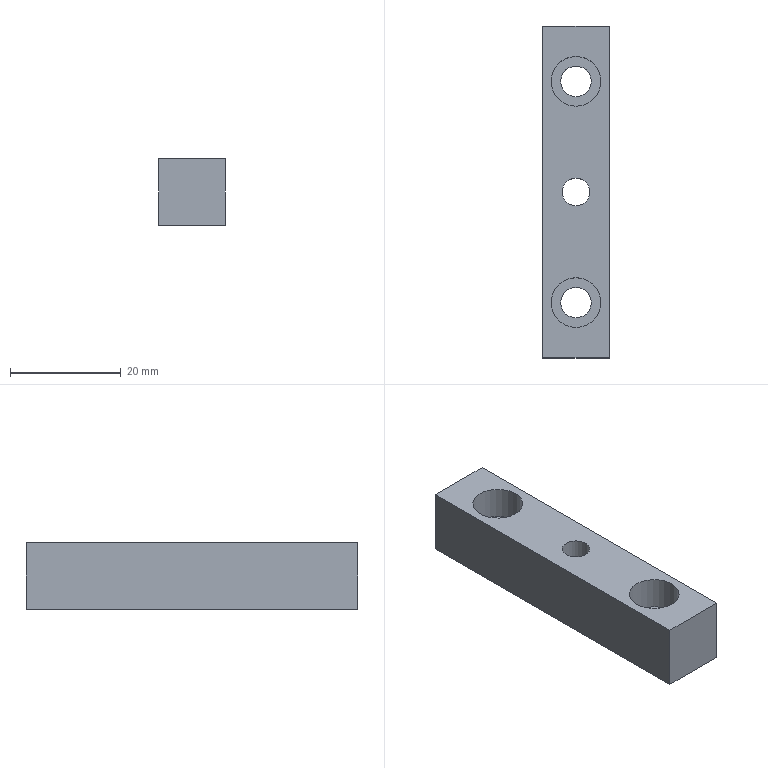Component | NX | COVER_PLATE | 1 solid | 13 faces | box 12 x 60 x 12 mm | volume 7356 mm3 | plane 8 | cylinder 5 | commonest cylinder face diameters 5.5 x2 9 x2 5 x1
STEP:
#1=CARTESIAN_POINT('',(0.,0.,0.));
#2=DIRECTION('',(0.,0.,1.));
#3=DIRECTION('',(1.,0.,0.));
#4=AXIS2_PLACEMENT_3D('',#1,#2,#3);
#5=CARTESIAN_POINT('',(0.,17.25,53.5));
#6=VERTEX_POINT('',#5);
#7=CARTESIAN_POINT('',(0.,20.,53.5));
#8=DIRECTION('',(0.,0.,-1.));
#9=DIRECTION('',(0.,-1.,0.));
#10=AXIS2_PLACEMENT_3D('',#7,#8,#9);
#11=CIRCLE('',#10,2.75);
#12=CARTESIAN_POINT('',(0.,20.,65.5));
#13=DIRECTION('',(0.,0.,-1.));
#14=DIRECTION('',(0.,1.,0.));
#15=AXIS2_PLACEMENT_3D('',#12,#13,#14);
#16=CYLINDRICAL_SURFACE('',#15,2.75);
#17=CARTESIAN_POINT('',(3.142,12.));
#18=DIRECTION('',(1.,0.));
#19=VECTOR('',#18,1.);
#20=LINE('',#17,#19);
#21=(GEOMETRIC_REPRESENTATION_CONTEXT(2)PARAMETRIC_REPRESENTATION_CONTEXT()REPRESENTATION_CONTEXT('',''));
#22=DEFINITIONAL_REPRESENTATION('',(#20),#21);
#23=PCURVE('',#16,#22);
#24=CARTESIAN_POINT('',(0.,-0.,53.5));
#25=DIRECTION('',(0.,0.,1.));
#26=DIRECTION('',(0.,-1.,0.));
#27=AXIS2_PLACEMENT_3D('',#24,#25,#26);
#28=PLANE('',#27);
#29=CARTESIAN_POINT('',(-17.25,-0.));
#30=CARTESIAN_POINT('',(-17.25,-4.763));
#31=CARTESIAN_POINT('',(-21.375,-2.382));
#32=CARTESIAN_POINT('',(-25.5,-0.));
#33=CARTESIAN_POINT('',(-21.375,2.382));
#34=CARTESIAN_POINT('',(-17.25,4.763));
#35=CARTESIAN_POINT('',(-17.25,-0.));
#36=(BOUNDED_CURVE()B_SPLINE_CURVE(2,(#29,#30,#31,#32,#33,#34,#35),.UNSPECIFIED.,.T.,.F.)B_SPLINE_CURVE_WITH_KNOTS((1,2,2,2,2,1),(-2.094,0.,2.094,4.189,6.283,8.378),.UNSPECIFIED.)CURVE()GEOMETRIC_REPRESENTATION_ITEM()RATIONAL_B_SPLINE_CURVE((1.,0.5,1.,0.5,1.,0.5,1.))REPRESENTATION_ITEM(''));
#37=(GEOMETRIC_REPRESENTATION_CONTEXT(2)PARAMETRIC_REPRESENTATION_CONTEXT()REPRESENTATION_CONTEXT('',''));
#38=DEFINITIONAL_REPRESENTATION('',(#36),#37);
#39=PCURVE('',#28,#38);
#40=SURFACE_CURVE('',#11,(#23,#39),.PCURVE_S1.);
#41=EDGE_CURVE('',#6,#6,#40,.T.);
#42=ORIENTED_EDGE('',*,*,#41,.F.);
#43=CARTESIAN_POINT('',(0.,17.25,59.5));
#44=VERTEX_POINT('',#43);
#45=CARTESIAN_POINT('',(0.,17.25,59.5));
#46=CARTESIAN_POINT('',(0.,17.25,53.5));
#47=B_SPLINE_CURVE_WITH_KNOTS('',1,(#45,#46),.UNSPECIFIED.,.F.,.F.,(2,2),(6.,12.),.PIECEWISE_BEZIER_KNOTS.);
#48=CARTESIAN_POINT('',(3.142,0.));
#49=DIRECTION('',(0.,1.));
#50=VECTOR('',#49,1.);
#51=LINE('',#48,#50);
#52=(GEOMETRIC_REPRESENTATION_CONTEXT(2)PARAMETRIC_REPRESENTATION_CONTEXT()REPRESENTATION_CONTEXT('',''));
#53=DEFINITIONAL_REPRESENTATION('',(#51),#52);
#54=PCURVE('',#16,#53);
#55=CARTESIAN_POINT('',(9.425,0.));
#56=DIRECTION('',(0.,1.));
#57=VECTOR('',#56,1.);
#58=LINE('',#55,#57);
#59=(GEOMETRIC_REPRESENTATION_CONTEXT(2)PARAMETRIC_REPRESENTATION_CONTEXT()REPRESENTATION_CONTEXT('',''));
#60=DEFINITIONAL_REPRESENTATION('',(#58),#59);
#61=PCURVE('',#16,#60);
#62=SEAM_CURVE('',#47,(#54,#61),.PCURVE_S1.);
#63=EDGE_CURVE('',#44,#6,#62,.T.);
#64=ORIENTED_EDGE('',*,*,#63,.F.);
#65=CARTESIAN_POINT('',(0.,20.,59.5));
#66=DIRECTION('',(0.,0.,-1.));
#67=DIRECTION('',(0.,-1.,0.));
#68=AXIS2_PLACEMENT_3D('',#65,#66,#67);
#69=CIRCLE('',#68,2.75);
#70=CARTESIAN_POINT('',(3.142,6.));
#71=DIRECTION('',(1.,0.));
#72=VECTOR('',#71,1.);
#73=LINE('',#70,#72);
#74=(GEOMETRIC_REPRESENTATION_CONTEXT(2)PARAMETRIC_REPRESENTATION_CONTEXT()REPRESENTATION_CONTEXT('',''));
#75=DEFINITIONAL_REPRESENTATION('',(#73),#74);
#76=PCURVE('',#16,#75);
#77=CARTESIAN_POINT('',(0.,20.,59.5));
#78=DIRECTION('',(0.,0.,1.));
#79=DIRECTION('',(0.,-1.,0.));
#80=AXIS2_PLACEMENT_3D('',#77,#78,#79);
#81=PLANE('',#80);
#82=CARTESIAN_POINT('',(2.75,0.));
#83=CARTESIAN_POINT('',(2.75,-4.763));
#84=CARTESIAN_POINT('',(-1.375,-2.382));
#85=CARTESIAN_POINT('',(-5.5,-0.));
#86=CARTESIAN_POINT('',(-1.375,2.382));
#87=CARTESIAN_POINT('',(2.75,4.763));
#88=CARTESIAN_POINT('',(2.75,0.));
#89=(BOUNDED_CURVE()B_SPLINE_CURVE(2,(#82,#83,#84,#85,#86,#87,#88),.UNSPECIFIED.,.T.,.F.)B_SPLINE_CURVE_WITH_KNOTS((1,2,2,2,2,1),(-2.094,0.,2.094,4.189,6.283,8.378),.UNSPECIFIED.)CURVE()GEOMETRIC_REPRESENTATION_ITEM()RATIONAL_B_SPLINE_CURVE((1.,0.5,1.,0.5,1.,0.5,1.))REPRESENTATION_ITEM(''));
#90=(GEOMETRIC_REPRESENTATION_CONTEXT(2)PARAMETRIC_REPRESENTATION_CONTEXT()REPRESENTATION_CONTEXT('',''));
#91=DEFINITIONAL_REPRESENTATION('',(#89),#90);
#92=PCURVE('',#81,#91);
#93=SURFACE_CURVE('',#69,(#76,#92),.PCURVE_S1.);
#94=EDGE_CURVE('',#44,#44,#93,.T.);
#95=ORIENTED_EDGE('',*,*,#94,.T.);
#96=ORIENTED_EDGE('',*,*,#63,.T.);
#97=EDGE_LOOP('',(#42,#64,#95,#96));
#98=FACE_BOUND('',#97,.F.);
#99=ADVANCED_FACE('',(#98),#16,.F.);
#100=CARTESIAN_POINT('',(0.,-17.25,53.5));
#101=VERTEX_POINT('',#100);
#102=CARTESIAN_POINT('',(0.,-20.,53.5));
#103=DIRECTION('',(0.,0.,-1.));
#104=DIRECTION('',(0.,1.,0.));
#105=AXIS2_PLACEMENT_3D('',#102,#103,#104);
#106=CIRCLE('',#105,2.75);
#107=CARTESIAN_POINT('',(0.,-20.,65.5));
#108=DIRECTION('',(0.,0.,-1.));
#109=DIRECTION('',(0.,1.,0.));
#110=AXIS2_PLACEMENT_3D('',#107,#108,#109);
#111=CYLINDRICAL_SURFACE('',#110,2.75);
#112=CARTESIAN_POINT('',(0.,12.));
#113=DIRECTION('',(1.,0.));
#114=VECTOR('',#113,1.);
#115=LINE('',#112,#114);
#116=(GEOMETRIC_REPRESENTATION_CONTEXT(2)PARAMETRIC_REPRESENTATION_CONTEXT()REPRESENTATION_CONTEXT('',''));
#117=DEFINITIONAL_REPRESENTATION('',(#115),#116);
#118=PCURVE('',#111,#117);
#119=CARTESIAN_POINT('',(17.25,-0.));
#120=CARTESIAN_POINT('',(17.25,4.763));
#121=CARTESIAN_POINT('',(21.375,2.382));
#122=CARTESIAN_POINT('',(25.5,-0.));
#123=CARTESIAN_POINT('',(21.375,-2.382));
#124=CARTESIAN_POINT('',(17.25,-4.763));
#125=CARTESIAN_POINT('',(17.25,-0.));
#126=(BOUNDED_CURVE()B_SPLINE_CURVE(2,(#119,#120,#121,#122,#123,#124,#125),.UNSPECIFIED.,.T.,.F.)B_SPLINE_CURVE_WITH_KNOTS((1,2,2,2,2,1),(-2.094,0.,2.094,4.189,6.283,8.378),.UNSPECIFIED.)CURVE()GEOMETRIC_REPRESENTATION_ITEM()RATIONAL_B_SPLINE_CURVE((1.,0.5,1.,0.5,1.,0.5,1.))REPRESENTATION_ITEM(''));
#127=(GEOMETRIC_REPRESENTATION_CONTEXT(2)PARAMETRIC_REPRESENTATION_CONTEXT()REPRESENTATION_CONTEXT('',''));
#128=DEFINITIONAL_REPRESENTATION('',(#126),#127);
#129=PCURVE('',#28,#128);
#130=SURFACE_CURVE('',#106,(#118,#129),.PCURVE_S1.);
#131=EDGE_CURVE('',#101,#101,#130,.T.);
#132=ORIENTED_EDGE('',*,*,#131,.F.);
#133=CARTESIAN_POINT('',(0.,-17.25,59.5));
#134=VERTEX_POINT('',#133);
#135=CARTESIAN_POINT('',(-0.,-17.25,59.5));
#136=CARTESIAN_POINT('',(-0.,-17.25,53.5));
#137=B_SPLINE_CURVE_WITH_KNOTS('',1,(#135,#136),.UNSPECIFIED.,.F.,.F.,(2,2),(6.,12.),.PIECEWISE_BEZIER_KNOTS.);
#138=CARTESIAN_POINT('',(0.,0.));
#139=DIRECTION('',(0.,1.));
#140=VECTOR('',#139,1.);
#141=LINE('',#138,#140);
#142=(GEOMETRIC_REPRESENTATION_CONTEXT(2)PARAMETRIC_REPRESENTATION_CONTEXT()REPRESENTATION_CONTEXT('',''));
#143=DEFINITIONAL_REPRESENTATION('',(#141),#142);
#144=PCURVE('',#111,#143);
#145=CARTESIAN_POINT('',(6.283,0.));
#146=DIRECTION('',(0.,1.));
#147=VECTOR('',#146,1.);
#148=LINE('',#145,#147);
#149=(GEOMETRIC_REPRESENTATION_CONTEXT(2)PARAMETRIC_REPRESENTATION_CONTEXT()REPRESENTATION_CONTEXT('',''));
#150=DEFINITIONAL_REPRESENTATION('',(#148),#149);
#151=PCURVE('',#111,#150);
#152=SEAM_CURVE('',#137,(#144,#151),.PCURVE_S1.);
#153=EDGE_CURVE('',#134,#101,#152,.T.);
#154=ORIENTED_EDGE('',*,*,#153,.F.);
#155=CARTESIAN_POINT('',(0.,-20.,59.5));
#156=DIRECTION('',(0.,0.,-1.));
#157=DIRECTION('',(0.,1.,0.));
#158=AXIS2_PLACEMENT_3D('',#155,#156,#157);
#159=CIRCLE('',#158,2.75);
#160=CARTESIAN_POINT('',(0.,6.));
#161=DIRECTION('',(1.,0.));
#162=VECTOR('',#161,1.);
#163=LINE('',#160,#162);
#164=(GEOMETRIC_REPRESENTATION_CONTEXT(2)PARAMETRIC_REPRESENTATION_CONTEXT()REPRESENTATION_CONTEXT('',''));
#165=DEFINITIONAL_REPRESENTATION('',(#163),#164);
#166=PCURVE('',#111,#165);
#167=CARTESIAN_POINT('',(0.,-20.,59.5));
#168=DIRECTION('',(0.,0.,1.));
#169=DIRECTION('',(0.,-1.,0.));
#170=AXIS2_PLACEMENT_3D('',#167,#168,#169);
#171=PLANE('',#170);
#172=CARTESIAN_POINT('',(-2.75,-0.));
#173=CARTESIAN_POINT('',(-2.75,4.763));
#174=CARTESIAN_POINT('',(1.375,2.382));
#175=CARTESIAN_POINT('',(5.5,0.));
#176=CARTESIAN_POINT('',(1.375,-2.382));
#177=CARTESIAN_POINT('',(-2.75,-4.763));
#178=CARTESIAN_POINT('',(-2.75,-0.));
#179=(BOUNDED_CURVE()B_SPLINE_CURVE(2,(#172,#173,#174,#175,#176,#177,#178),.UNSPECIFIED.,.T.,.F.)B_SPLINE_CURVE_WITH_KNOTS((1,2,2,2,2,1),(-2.094,0.,2.094,4.189,6.283,8.378),.UNSPECIFIED.)CURVE()GEOMETRIC_REPRESENTATION_ITEM()RATIONAL_B_SPLINE_CURVE((1.,0.5,1.,0.5,1.,0.5,1.))REPRESENTATION_ITEM(''));
#180=(GEOMETRIC_REPRESENTATION_CONTEXT(2)PARAMETRIC_REPRESENTATION_CONTEXT()REPRESENTATION_CONTEXT('',''));
#181=DEFINITIONAL_REPRESENTATION('',(#179),#180);
#182=PCURVE('',#171,#181);
#183=SURFACE_CURVE('',#159,(#166,#182),.PCURVE_S1.);
#184=EDGE_CURVE('',#134,#134,#183,.T.);
#185=ORIENTED_EDGE('',*,*,#184,.T.);
#186=ORIENTED_EDGE('',*,*,#153,.T.);
#187=EDGE_LOOP('',(#132,#154,#185,#186));
#188=FACE_BOUND('',#187,.F.);
#189=ADVANCED_FACE('',(#188),#111,.F.);
#190=CARTESIAN_POINT('',(6.,30.,53.5));
#191=VERTEX_POINT('',#190);
#192=CARTESIAN_POINT('',(-6.,30.,53.5));
#193=VERTEX_POINT('',#192);
#194=CARTESIAN_POINT('',(6.,30.,53.5));
#195=DIRECTION('',(-1.,0.,0.));
#196=VECTOR('',#195,1.);
#197=LINE('',#194,#196);
#198=CARTESIAN_POINT('',(6.,30.,65.5));
#199=DIRECTION('',(0.,-1.,0.));
#200=DIRECTION('',(0.,0.,-1.));
#201=AXIS2_PLACEMENT_3D('',#198,#199,#200);
#202=PLANE('',#201);
#203=CARTESIAN_POINT('',(12.,0.));
#204=DIRECTION('',(0.,-1.));
#205=VECTOR('',#204,1.);
#206=LINE('',#203,#205);
#207=(GEOMETRIC_REPRESENTATION_CONTEXT(2)PARAMETRIC_REPRESENTATION_CONTEXT()REPRESENTATION_CONTEXT('',''));
#208=DEFINITIONAL_REPRESENTATION('',(#206),#207);
#209=PCURVE('',#202,#208);
#210=CARTESIAN_POINT('',(-30.,6.));
#211=DIRECTION('',(0.,-1.));
#212=VECTOR('',#211,1.);
#213=LINE('',#210,#212);
#214=(GEOMETRIC_REPRESENTATION_CONTEXT(2)PARAMETRIC_REPRESENTATION_CONTEXT()REPRESENTATION_CONTEXT('',''));
#215=DEFINITIONAL_REPRESENTATION('',(#213),#214);
#216=PCURVE('',#28,#215);
#217=SURFACE_CURVE('',#197,(#209,#216),.PCURVE_S1.);
#218=EDGE_CURVE('',#191,#193,#217,.T.);
#219=ORIENTED_EDGE('',*,*,#218,.T.);
#220=CARTESIAN_POINT('',(-6.,30.,65.5));
#221=VERTEX_POINT('',#220);
#222=CARTESIAN_POINT('',(-6.,30.,65.5));
#223=DIRECTION('',(0.,0.,-1.));
#224=VECTOR('',#223,1.);
#225=LINE('',#222,#224);
#226=CARTESIAN_POINT('',(0.,-12.));
#227=DIRECTION('',(1.,0.));
#228=VECTOR('',#227,1.);
#229=LINE('',#226,#228);
#230=(GEOMETRIC_REPRESENTATION_CONTEXT(2)PARAMETRIC_REPRESENTATION_CONTEXT()REPRESENTATION_CONTEXT('',''));
#231=DEFINITIONAL_REPRESENTATION('',(#229),#230);
#232=PCURVE('',#202,#231);
#233=CARTESIAN_POINT('',(-6.,30.,65.5));
#234=DIRECTION('',(1.,0.,0.));
#235=DIRECTION('',(0.,0.,1.));
#236=AXIS2_PLACEMENT_3D('',#233,#234,#235);
#237=PLANE('',#236);
#238=CARTESIAN_POINT('',(0.,0.));
#239=DIRECTION('',(-1.,0.));
#240=VECTOR('',#239,1.);
#241=LINE('',#238,#240);
#242=(GEOMETRIC_REPRESENTATION_CONTEXT(2)PARAMETRIC_REPRESENTATION_CONTEXT()REPRESENTATION_CONTEXT('',''));
#243=DEFINITIONAL_REPRESENTATION('',(#241),#242);
#244=PCURVE('',#237,#243);
#245=SURFACE_CURVE('',#225,(#232,#244),.PCURVE_S1.);
#246=EDGE_CURVE('',#221,#193,#245,.T.);
#247=ORIENTED_EDGE('',*,*,#246,.F.);
#248=CARTESIAN_POINT('',(6.,30.,65.5));
#249=VERTEX_POINT('',#248);
#250=CARTESIAN_POINT('',(6.,30.,65.5));
#251=DIRECTION('',(-1.,0.,0.));
#252=VECTOR('',#251,1.);
#253=LINE('',#250,#252);
#254=CARTESIAN_POINT('',(0.,0.));
#255=DIRECTION('',(0.,-1.));
#256=VECTOR('',#255,1.);
#257=LINE('',#254,#256);
#258=(GEOMETRIC_REPRESENTATION_CONTEXT(2)PARAMETRIC_REPRESENTATION_CONTEXT()REPRESENTATION_CONTEXT('',''));
#259=DEFINITIONAL_REPRESENTATION('',(#257),#258);
#260=PCURVE('',#202,#259);
#261=CARTESIAN_POINT('',(0.,-0.,65.5));
#262=DIRECTION('',(0.,0.,1.));
#263=DIRECTION('',(0.,-1.,0.));
#264=AXIS2_PLACEMENT_3D('',#261,#262,#263);
#265=PLANE('',#264);
#266=CARTESIAN_POINT('',(-30.,6.));
#267=DIRECTION('',(0.,-1.));
#268=VECTOR('',#267,1.);
#269=LINE('',#266,#268);
#270=(GEOMETRIC_REPRESENTATION_CONTEXT(2)PARAMETRIC_REPRESENTATION_CONTEXT()REPRESENTATION_CONTEXT('',''));
#271=DEFINITIONAL_REPRESENTATION('',(#269),#270);
#272=PCURVE('',#265,#271);
#273=SURFACE_CURVE('',#253,(#260,#272),.PCURVE_S1.);
#274=EDGE_CURVE('',#249,#221,#273,.T.);
#275=ORIENTED_EDGE('',*,*,#274,.F.);
#276=CARTESIAN_POINT('',(6.,30.,65.5));
#277=DIRECTION('',(0.,0.,-1.));
#278=VECTOR('',#277,1.);
#279=LINE('',#276,#278);
#280=CARTESIAN_POINT('',(0.,0.));
#281=DIRECTION('',(1.,0.));
#282=VECTOR('',#281,1.);
#283=LINE('',#280,#282);
#284=(GEOMETRIC_REPRESENTATION_CONTEXT(2)PARAMETRIC_REPRESENTATION_CONTEXT()REPRESENTATION_CONTEXT('',''));
#285=DEFINITIONAL_REPRESENTATION('',(#283),#284);
#286=PCURVE('',#202,#285);
#287=CARTESIAN_POINT('',(6.,-30.,65.5));
#288=DIRECTION('',(-1.,0.,0.));
#289=DIRECTION('',(0.,0.,-1.));
#290=AXIS2_PLACEMENT_3D('',#287,#288,#289);
#291=PLANE('',#290);
#292=CARTESIAN_POINT('',(0.,-60.));
#293=DIRECTION('',(1.,0.));
#294=VECTOR('',#293,1.);
#295=LINE('',#292,#294);
#296=(GEOMETRIC_REPRESENTATION_CONTEXT(2)PARAMETRIC_REPRESENTATION_CONTEXT()REPRESENTATION_CONTEXT('',''));
#297=DEFINITIONAL_REPRESENTATION('',(#295),#296);
#298=PCURVE('',#291,#297);
#299=SURFACE_CURVE('',#279,(#286,#298),.PCURVE_S1.);
#300=EDGE_CURVE('',#249,#191,#299,.T.);
#301=ORIENTED_EDGE('',*,*,#300,.T.);
#302=EDGE_LOOP('',(#219,#247,#275,#301));
#303=FACE_BOUND('',#302,.T.);
#304=ADVANCED_FACE('',(#303),#202,.F.);
#305=CARTESIAN_POINT('',(-6.,-30.,53.5));
#306=VERTEX_POINT('',#305);
#307=CARTESIAN_POINT('',(-6.,30.,53.5));
#308=DIRECTION('',(0.,-1.,0.));
#309=VECTOR('',#308,1.);
#310=LINE('',#307,#309);
#311=CARTESIAN_POINT('',(-12.,0.));
#312=DIRECTION('',(0.,1.));
#313=VECTOR('',#312,1.);
#314=LINE('',#311,#313);
#315=(GEOMETRIC_REPRESENTATION_CONTEXT(2)PARAMETRIC_REPRESENTATION_CONTEXT()REPRESENTATION_CONTEXT('',''));
#316=DEFINITIONAL_REPRESENTATION('',(#314),#315);
#317=PCURVE('',#237,#316);
#318=CARTESIAN_POINT('',(-30.,-6.));
#319=DIRECTION('',(1.,0.));
#320=VECTOR('',#319,1.);
#321=LINE('',#318,#320);
#322=(GEOMETRIC_REPRESENTATION_CONTEXT(2)PARAMETRIC_REPRESENTATION_CONTEXT()REPRESENTATION_CONTEXT('',''));
#323=DEFINITIONAL_REPRESENTATION('',(#321),#322);
#324=PCURVE('',#28,#323);
#325=SURFACE_CURVE('',#310,(#317,#324),.PCURVE_S1.);
#326=EDGE_CURVE('',#193,#306,#325,.T.);
#327=ORIENTED_EDGE('',*,*,#326,.T.);
#328=CARTESIAN_POINT('',(-6.,-30.,65.5));
#329=VERTEX_POINT('',#328);
#330=CARTESIAN_POINT('',(-6.,-30.,65.5));
#331=DIRECTION('',(0.,0.,-1.));
#332=VECTOR('',#331,1.);
#333=LINE('',#330,#332);
#334=CARTESIAN_POINT('',(0.,60.));
#335=DIRECTION('',(-1.,0.));
#336=VECTOR('',#335,1.);
#337=LINE('',#334,#336);
#338=(GEOMETRIC_REPRESENTATION_CONTEXT(2)PARAMETRIC_REPRESENTATION_CONTEXT()REPRESENTATION_CONTEXT('',''));
#339=DEFINITIONAL_REPRESENTATION('',(#337),#338);
#340=PCURVE('',#237,#339);
#341=CARTESIAN_POINT('',(-6.,-30.,65.5));
#342=DIRECTION('',(0.,1.,0.));
#343=DIRECTION('',(0.,0.,1.));
#344=AXIS2_PLACEMENT_3D('',#341,#342,#343);
#345=PLANE('',#344);
#346=CARTESIAN_POINT('',(0.,0.));
#347=DIRECTION('',(-1.,0.));
#348=VECTOR('',#347,1.);
#349=LINE('',#346,#348);
#350=(GEOMETRIC_REPRESENTATION_CONTEXT(2)PARAMETRIC_REPRESENTATION_CONTEXT()REPRESENTATION_CONTEXT('',''));
#351=DEFINITIONAL_REPRESENTATION('',(#349),#350);
#352=PCURVE('',#345,#351);
#353=SURFACE_CURVE('',#333,(#340,#352),.PCURVE_S1.);
#354=EDGE_CURVE('',#329,#306,#353,.T.);
#355=ORIENTED_EDGE('',*,*,#354,.F.);
#356=CARTESIAN_POINT('',(-6.,30.,65.5));
#357=DIRECTION('',(0.,-1.,0.));
#358=VECTOR('',#357,1.);
#359=LINE('',#356,#358);
#360=CARTESIAN_POINT('',(0.,0.));
#361=DIRECTION('',(0.,1.));
#362=VECTOR('',#361,1.);
#363=LINE('',#360,#362);
#364=(GEOMETRIC_REPRESENTATION_CONTEXT(2)PARAMETRIC_REPRESENTATION_CONTEXT()REPRESENTATION_CONTEXT('',''));
#365=DEFINITIONAL_REPRESENTATION('',(#363),#364);
#366=PCURVE('',#237,#365);
#367=CARTESIAN_POINT('',(-30.,-6.));
#368=DIRECTION('',(1.,0.));
#369=VECTOR('',#368,1.);
#370=LINE('',#367,#369);
#371=(GEOMETRIC_REPRESENTATION_CONTEXT(2)PARAMETRIC_REPRESENTATION_CONTEXT()REPRESENTATION_CONTEXT('',''));
#372=DEFINITIONAL_REPRESENTATION('',(#370),#371);
#373=PCURVE('',#265,#372);
#374=SURFACE_CURVE('',#359,(#366,#373),.PCURVE_S1.);
#375=EDGE_CURVE('',#221,#329,#374,.T.);
#376=ORIENTED_EDGE('',*,*,#375,.F.);
#377=ORIENTED_EDGE('',*,*,#246,.T.);
#378=EDGE_LOOP('',(#327,#355,#376,#377));
#379=FACE_BOUND('',#378,.T.);
#380=ADVANCED_FACE('',(#379),#237,.F.);
#381=CARTESIAN_POINT('',(6.,-30.,53.5));
#382=VERTEX_POINT('',#381);
#383=CARTESIAN_POINT('',(-6.,-30.,53.5));
#384=DIRECTION('',(1.,0.,0.));
#385=VECTOR('',#384,1.);
#386=LINE('',#383,#385);
#387=CARTESIAN_POINT('',(-12.,0.));
#388=DIRECTION('',(0.,1.));
#389=VECTOR('',#388,1.);
#390=LINE('',#387,#389);
#391=(GEOMETRIC_REPRESENTATION_CONTEXT(2)PARAMETRIC_REPRESENTATION_CONTEXT()REPRESENTATION_CONTEXT('',''));
#392=DEFINITIONAL_REPRESENTATION('',(#390),#391);
#393=PCURVE('',#345,#392);
#394=CARTESIAN_POINT('',(30.,-6.));
#395=DIRECTION('',(0.,1.));
#396=VECTOR('',#395,1.);
#397=LINE('',#394,#396);
#398=(GEOMETRIC_REPRESENTATION_CONTEXT(2)PARAMETRIC_REPRESENTATION_CONTEXT()REPRESENTATION_CONTEXT('',''));
#399=DEFINITIONAL_REPRESENTATION('',(#397),#398);
#400=PCURVE('',#28,#399);
#401=SURFACE_CURVE('',#386,(#393,#400),.PCURVE_S1.);
#402=EDGE_CURVE('',#306,#382,#401,.T.);
#403=ORIENTED_EDGE('',*,*,#402,.T.);
#404=CARTESIAN_POINT('',(6.,-30.,65.5));
#405=VERTEX_POINT('',#404);
#406=CARTESIAN_POINT('',(6.,-30.,65.5));
#407=DIRECTION('',(0.,0.,-1.));
#408=VECTOR('',#407,1.);
#409=LINE('',#406,#408);
#410=CARTESIAN_POINT('',(0.,12.));
#411=DIRECTION('',(-1.,0.));
#412=VECTOR('',#411,1.);
#413=LINE('',#410,#412);
#414=(GEOMETRIC_REPRESENTATION_CONTEXT(2)PARAMETRIC_REPRESENTATION_CONTEXT()REPRESENTATION_CONTEXT('',''));
#415=DEFINITIONAL_REPRESENTATION('',(#413),#414);
#416=PCURVE('',#345,#415);
#417=CARTESIAN_POINT('',(0.,0.));
#418=DIRECTION('',(1.,0.));
#419=VECTOR('',#418,1.);
#420=LINE('',#417,#419);
#421=(GEOMETRIC_REPRESENTATION_CONTEXT(2)PARAMETRIC_REPRESENTATION_CONTEXT()REPRESENTATION_CONTEXT('',''));
#422=DEFINITIONAL_REPRESENTATION('',(#420),#421);
#423=PCURVE('',#291,#422);
#424=SURFACE_CURVE('',#409,(#416,#423),.PCURVE_S1.);
#425=EDGE_CURVE('',#405,#382,#424,.T.);
#426=ORIENTED_EDGE('',*,*,#425,.F.);
#427=CARTESIAN_POINT('',(-6.,-30.,65.5));
#428=DIRECTION('',(1.,0.,0.));
#429=VECTOR('',#428,1.);
#430=LINE('',#427,#429);
#431=CARTESIAN_POINT('',(0.,0.));
#432=DIRECTION('',(0.,1.));
#433=VECTOR('',#432,1.);
#434=LINE('',#431,#433);
#435=(GEOMETRIC_REPRESENTATION_CONTEXT(2)PARAMETRIC_REPRESENTATION_CONTEXT()REPRESENTATION_CONTEXT('',''));
#436=DEFINITIONAL_REPRESENTATION('',(#434),#435);
#437=PCURVE('',#345,#436);
#438=CARTESIAN_POINT('',(30.,-6.));
#439=DIRECTION('',(0.,1.));
#440=VECTOR('',#439,1.);
#441=LINE('',#438,#440);
#442=(GEOMETRIC_REPRESENTATION_CONTEXT(2)PARAMETRIC_REPRESENTATION_CONTEXT()REPRESENTATION_CONTEXT('',''));
#443=DEFINITIONAL_REPRESENTATION('',(#441),#442);
#444=PCURVE('',#265,#443);
#445=SURFACE_CURVE('',#430,(#437,#444),.PCURVE_S1.);
#446=EDGE_CURVE('',#329,#405,#445,.T.);
#447=ORIENTED_EDGE('',*,*,#446,.F.);
#448=ORIENTED_EDGE('',*,*,#354,.T.);
#449=EDGE_LOOP('',(#403,#426,#447,#448));
#450=FACE_BOUND('',#449,.T.);
#451=ADVANCED_FACE('',(#450),#345,.F.);
#452=CARTESIAN_POINT('',(6.,-30.,53.5));
#453=DIRECTION('',(0.,1.,0.));
#454=VECTOR('',#453,1.);
#455=LINE('',#452,#454);
#456=CARTESIAN_POINT('',(12.,0.));
#457=DIRECTION('',(0.,-1.));
#458=VECTOR('',#457,1.);
#459=LINE('',#456,#458);
#460=(GEOMETRIC_REPRESENTATION_CONTEXT(2)PARAMETRIC_REPRESENTATION_CONTEXT()REPRESENTATION_CONTEXT('',''));
#461=DEFINITIONAL_REPRESENTATION('',(#459),#460);
#462=PCURVE('',#291,#461);
#463=CARTESIAN_POINT('',(30.,6.));
#464=DIRECTION('',(-1.,0.));
#465=VECTOR('',#464,1.);
#466=LINE('',#463,#465);
#467=(GEOMETRIC_REPRESENTATION_CONTEXT(2)PARAMETRIC_REPRESENTATION_CONTEXT()REPRESENTATION_CONTEXT('',''));
#468=DEFINITIONAL_REPRESENTATION('',(#466),#467);
#469=PCURVE('',#28,#468);
#470=SURFACE_CURVE('',#455,(#462,#469),.PCURVE_S1.);
#471=EDGE_CURVE('',#382,#191,#470,.T.);
#472=ORIENTED_EDGE('',*,*,#471,.T.);
#473=ORIENTED_EDGE('',*,*,#300,.F.);
#474=CARTESIAN_POINT('',(6.,-30.,65.5));
#475=DIRECTION('',(0.,1.,0.));
#476=VECTOR('',#475,1.);
#477=LINE('',#474,#476);
#478=CARTESIAN_POINT('',(0.,0.));
#479=DIRECTION('',(0.,-1.));
#480=VECTOR('',#479,1.);
#481=LINE('',#478,#480);
#482=(GEOMETRIC_REPRESENTATION_CONTEXT(2)PARAMETRIC_REPRESENTATION_CONTEXT()REPRESENTATION_CONTEXT('',''));
#483=DEFINITIONAL_REPRESENTATION('',(#481),#482);
#484=PCURVE('',#291,#483);
#485=CARTESIAN_POINT('',(30.,6.));
#486=DIRECTION('',(-1.,0.));
#487=VECTOR('',#486,1.);
#488=LINE('',#485,#487);
#489=(GEOMETRIC_REPRESENTATION_CONTEXT(2)PARAMETRIC_REPRESENTATION_CONTEXT()REPRESENTATION_CONTEXT('',''));
#490=DEFINITIONAL_REPRESENTATION('',(#488),#489);
#491=PCURVE('',#265,#490);
#492=SURFACE_CURVE('',#477,(#484,#491),.PCURVE_S1.);
#493=EDGE_CURVE('',#405,#249,#492,.T.);
#494=ORIENTED_EDGE('',*,*,#493,.F.);
#495=ORIENTED_EDGE('',*,*,#425,.T.);
#496=EDGE_LOOP('',(#472,#473,#494,#495));
#497=FACE_BOUND('',#496,.T.);
#498=ADVANCED_FACE('',(#497),#291,.F.);
#499=CARTESIAN_POINT('',(0.,-15.5,65.5));
#500=VERTEX_POINT('',#499);
#501=CARTESIAN_POINT('',(0.,-20.,65.5));
#502=DIRECTION('',(0.,0.,1.));
#503=DIRECTION('',(0.,1.,0.));
#504=AXIS2_PLACEMENT_3D('',#501,#502,#503);
#505=CIRCLE('',#504,4.5);
#506=CARTESIAN_POINT('',(20.,0.));
#507=DIRECTION('',(-1.,0.));
#508=AXIS2_PLACEMENT_2D('',#506,#507);
#509=CIRCLE('',#508,4.5);
#510=(GEOMETRIC_REPRESENTATION_CONTEXT(2)PARAMETRIC_REPRESENTATION_CONTEXT()REPRESENTATION_CONTEXT('',''));
#511=DEFINITIONAL_REPRESENTATION('',(#509),#510);
#512=PCURVE('',#265,#511);
#513=CARTESIAN_POINT('',(0.,-20.,59.5));
#514=DIRECTION('',(0.,0.,1.));
#515=DIRECTION('',(0.,-1.,0.));
#516=AXIS2_PLACEMENT_3D('',#513,#514,#515);
#517=CYLINDRICAL_SURFACE('',#516,4.5);
#518=CARTESIAN_POINT('',(3.142,6.));
#519=DIRECTION('',(1.,0.));
#520=VECTOR('',#519,1.);
#521=LINE('',#518,#520);
#522=(GEOMETRIC_REPRESENTATION_CONTEXT(2)PARAMETRIC_REPRESENTATION_CONTEXT()REPRESENTATION_CONTEXT('',''));
#523=DEFINITIONAL_REPRESENTATION('',(#521),#522);
#524=PCURVE('',#517,#523);
#525=SURFACE_CURVE('',#505,(#512,#524),.PCURVE_S1.);
#526=EDGE_CURVE('',#500,#500,#525,.T.);
#527=ORIENTED_EDGE('',*,*,#526,.F.);
#528=EDGE_LOOP('',(#527));
#529=FACE_BOUND('',#528,.T.);
#530=CARTESIAN_POINT('',(0.,15.5,65.5));
#531=VERTEX_POINT('',#530);
#532=CARTESIAN_POINT('',(0.,20.,65.5));
#533=DIRECTION('',(0.,0.,1.));
#534=DIRECTION('',(0.,-1.,0.));
#535=AXIS2_PLACEMENT_3D('',#532,#533,#534);
#536=CIRCLE('',#535,4.5);
#537=CARTESIAN_POINT('',(-20.,0.));
#538=DIRECTION('',(1.,0.));
#539=AXIS2_PLACEMENT_2D('',#537,#538);
#540=CIRCLE('',#539,4.5);
#541=(GEOMETRIC_REPRESENTATION_CONTEXT(2)PARAMETRIC_REPRESENTATION_CONTEXT()REPRESENTATION_CONTEXT('',''));
#542=DEFINITIONAL_REPRESENTATION('',(#540),#541);
#543=PCURVE('',#265,#542);
#544=CARTESIAN_POINT('',(0.,20.,59.5));
#545=DIRECTION('',(0.,0.,1.));
#546=DIRECTION('',(0.,-1.,0.));
#547=AXIS2_PLACEMENT_3D('',#544,#545,#546);
#548=CYLINDRICAL_SURFACE('',#547,4.5);
#549=CARTESIAN_POINT('',(0.,6.));
#550=DIRECTION('',(1.,0.));
#551=VECTOR('',#550,1.);
#552=LINE('',#549,#551);
#553=(GEOMETRIC_REPRESENTATION_CONTEXT(2)PARAMETRIC_REPRESENTATION_CONTEXT()REPRESENTATION_CONTEXT('',''));
#554=DEFINITIONAL_REPRESENTATION('',(#552),#553);
#555=PCURVE('',#548,#554);
#556=SURFACE_CURVE('',#536,(#543,#555),.PCURVE_S1.);
#557=EDGE_CURVE('',#531,#531,#556,.T.);
#558=ORIENTED_EDGE('',*,*,#557,.F.);
#559=EDGE_LOOP('',(#558));
#560=FACE_BOUND('',#559,.T.);
#561=CARTESIAN_POINT('',(0.,-2.5,65.5));
#562=VERTEX_POINT('',#561);
#563=CARTESIAN_POINT('',(0.,-0.,65.5));
#564=DIRECTION('',(0.,0.,-1.));
#565=DIRECTION('',(0.,-1.,0.));
#566=AXIS2_PLACEMENT_3D('',#563,#564,#565);
#567=CIRCLE('',#566,2.5);
#568=CARTESIAN_POINT('',(2.5,0.));
#569=CARTESIAN_POINT('',(2.5,-4.33));
#570=CARTESIAN_POINT('',(-1.25,-2.165));
#571=CARTESIAN_POINT('',(-5.,-0.));
#572=CARTESIAN_POINT('',(-1.25,2.165));
#573=CARTESIAN_POINT('',(2.5,4.33));
#574=CARTESIAN_POINT('',(2.5,0.));
#575=(BOUNDED_CURVE()B_SPLINE_CURVE(2,(#568,#569,#570,#571,#572,#573,#574),.UNSPECIFIED.,.T.,.F.)B_SPLINE_CURVE_WITH_KNOTS((1,2,2,2,2,1),(-2.094,0.,2.094,4.189,6.283,8.378),.UNSPECIFIED.)CURVE()GEOMETRIC_REPRESENTATION_ITEM()RATIONAL_B_SPLINE_CURVE((1.,0.5,1.,0.5,1.,0.5,1.))REPRESENTATION_ITEM(''));
#576=(GEOMETRIC_REPRESENTATION_CONTEXT(2)PARAMETRIC_REPRESENTATION_CONTEXT()REPRESENTATION_CONTEXT('',''));
#577=DEFINITIONAL_REPRESENTATION('',(#575),#576);
#578=PCURVE('',#265,#577);
#579=CARTESIAN_POINT('',(0.,-0.,65.5));
#580=DIRECTION('',(0.,0.,-1.));
#581=DIRECTION('',(0.,1.,0.));
#582=AXIS2_PLACEMENT_3D('',#579,#580,#581);
#583=CYLINDRICAL_SURFACE('',#582,2.5);
#584=CARTESIAN_POINT('',(3.142,0.));
#585=DIRECTION('',(1.,0.));
#586=VECTOR('',#585,1.);
#587=LINE('',#584,#586);
#588=(GEOMETRIC_REPRESENTATION_CONTEXT(2)PARAMETRIC_REPRESENTATION_CONTEXT()REPRESENTATION_CONTEXT('',''));
#589=DEFINITIONAL_REPRESENTATION('',(#587),#588);
#590=PCURVE('',#583,#589);
#591=SURFACE_CURVE('',#567,(#578,#590),.PCURVE_S1.);
#592=EDGE_CURVE('',#562,#562,#591,.T.);
#593=ORIENTED_EDGE('',*,*,#592,.T.);
#594=EDGE_LOOP('',(#593));
#595=FACE_BOUND('',#594,.T.);
#596=ORIENTED_EDGE('',*,*,#274,.T.);
#597=ORIENTED_EDGE('',*,*,#375,.T.);
#598=ORIENTED_EDGE('',*,*,#446,.T.);
#599=ORIENTED_EDGE('',*,*,#493,.T.);
#600=EDGE_LOOP('',(#596,#597,#598,#599));
#601=FACE_BOUND('',#600,.T.);
#602=ADVANCED_FACE('',(#529,#560,#595,#601),#265,.T.);
#603=ORIENTED_EDGE('',*,*,#131,.F.);
#604=EDGE_LOOP('',(#603));
#605=FACE_BOUND('',#604,.T.);
#606=ORIENTED_EDGE('',*,*,#41,.F.);
#607=EDGE_LOOP('',(#606));
#608=FACE_BOUND('',#607,.T.);
#609=CARTESIAN_POINT('',(0.,-2.5,53.5));
#610=VERTEX_POINT('',#609);
#611=CARTESIAN_POINT('',(0.,-0.,53.5));
#612=DIRECTION('',(0.,0.,-1.));
#613=DIRECTION('',(0.,-1.,0.));
#614=AXIS2_PLACEMENT_3D('',#611,#612,#613);
#615=CIRCLE('',#614,2.5);
#616=CARTESIAN_POINT('',(2.5,0.));
#617=CARTESIAN_POINT('',(2.5,-4.33));
#618=CARTESIAN_POINT('',(-1.25,-2.165));
#619=CARTESIAN_POINT('',(-5.,-0.));
#620=CARTESIAN_POINT('',(-1.25,2.165));
#621=CARTESIAN_POINT('',(2.5,4.33));
#622=CARTESIAN_POINT('',(2.5,0.));
#623=(BOUNDED_CURVE()B_SPLINE_CURVE(2,(#616,#617,#618,#619,#620,#621,#622),.UNSPECIFIED.,.T.,.F.)B_SPLINE_CURVE_WITH_KNOTS((1,2,2,2,2,1),(-2.094,0.,2.094,4.189,6.283,8.378),.UNSPECIFIED.)CURVE()GEOMETRIC_REPRESENTATION_ITEM()RATIONAL_B_SPLINE_CURVE((1.,0.5,1.,0.5,1.,0.5,1.))REPRESENTATION_ITEM(''));
#624=(GEOMETRIC_REPRESENTATION_CONTEXT(2)PARAMETRIC_REPRESENTATION_CONTEXT()REPRESENTATION_CONTEXT('',''));
#625=DEFINITIONAL_REPRESENTATION('',(#623),#624);
#626=PCURVE('',#28,#625);
#627=CARTESIAN_POINT('',(3.142,12.));
#628=DIRECTION('',(1.,0.));
#629=VECTOR('',#628,1.);
#630=LINE('',#627,#629);
#631=(GEOMETRIC_REPRESENTATION_CONTEXT(2)PARAMETRIC_REPRESENTATION_CONTEXT()REPRESENTATION_CONTEXT('',''));
#632=DEFINITIONAL_REPRESENTATION('',(#630),#631);
#633=PCURVE('',#583,#632);
#634=SURFACE_CURVE('',#615,(#626,#633),.PCURVE_S1.);
#635=EDGE_CURVE('',#610,#610,#634,.T.);
#636=ORIENTED_EDGE('',*,*,#635,.F.);
#637=EDGE_LOOP('',(#636));
#638=FACE_BOUND('',#637,.T.);
#639=ORIENTED_EDGE('',*,*,#218,.F.);
#640=ORIENTED_EDGE('',*,*,#471,.F.);
#641=ORIENTED_EDGE('',*,*,#402,.F.);
#642=ORIENTED_EDGE('',*,*,#326,.F.);
#643=EDGE_LOOP('',(#639,#640,#641,#642));
#644=FACE_BOUND('',#643,.T.);
#645=ADVANCED_FACE('',(#605,#608,#638,#644),#28,.F.);
#646=ORIENTED_EDGE('',*,*,#592,.T.);
#647=CARTESIAN_POINT('',(0.,-2.5,65.5));
#648=CARTESIAN_POINT('',(0.,-2.5,53.5));
#649=B_SPLINE_CURVE_WITH_KNOTS('',1,(#647,#648),.UNSPECIFIED.,.F.,.F.,(2,2),(0.,12.),.PIECEWISE_BEZIER_KNOTS.);
#650=CARTESIAN_POINT('',(9.425,0.));
#651=DIRECTION('',(0.,1.));
#652=VECTOR('',#651,1.);
#653=LINE('',#650,#652);
#654=(GEOMETRIC_REPRESENTATION_CONTEXT(2)PARAMETRIC_REPRESENTATION_CONTEXT()REPRESENTATION_CONTEXT('',''));
#655=DEFINITIONAL_REPRESENTATION('',(#653),#654);
#656=PCURVE('',#583,#655);
#657=CARTESIAN_POINT('',(3.142,0.));
#658=DIRECTION('',(0.,1.));
#659=VECTOR('',#658,1.);
#660=LINE('',#657,#659);
#661=(GEOMETRIC_REPRESENTATION_CONTEXT(2)PARAMETRIC_REPRESENTATION_CONTEXT()REPRESENTATION_CONTEXT('',''));
#662=DEFINITIONAL_REPRESENTATION('',(#660),#661);
#663=PCURVE('',#583,#662);
#664=SEAM_CURVE('',#649,(#656,#663),.PCURVE_S1.);
#665=EDGE_CURVE('',#562,#610,#664,.T.);
#666=ORIENTED_EDGE('',*,*,#665,.T.);
#667=ORIENTED_EDGE('',*,*,#635,.F.);
#668=ORIENTED_EDGE('',*,*,#665,.F.);
#669=EDGE_LOOP('',(#646,#666,#667,#668));
#670=FACE_BOUND('',#669,.F.);
#671=ADVANCED_FACE('',(#670),#583,.F.);
#672=CARTESIAN_POINT('',(0.,-15.5,59.5));
#673=VERTEX_POINT('',#672);
#674=CARTESIAN_POINT('',(0.,-20.,59.5));
#675=DIRECTION('',(0.,0.,-1.));
#676=DIRECTION('',(0.,1.,0.));
#677=AXIS2_PLACEMENT_3D('',#674,#675,#676);
#678=CIRCLE('',#677,4.5);
#679=CARTESIAN_POINT('',(9.425,0.));
#680=DIRECTION('',(-1.,0.));
#681=VECTOR('',#680,1.);
#682=LINE('',#679,#681);
#683=(GEOMETRIC_REPRESENTATION_CONTEXT(2)PARAMETRIC_REPRESENTATION_CONTEXT()REPRESENTATION_CONTEXT('',''));
#684=DEFINITIONAL_REPRESENTATION('',(#682),#683);
#685=PCURVE('',#517,#684);
#686=CARTESIAN_POINT('',(-4.5,0.));
#687=CARTESIAN_POINT('',(-4.5,7.794));
#688=CARTESIAN_POINT('',(2.25,3.897));
#689=CARTESIAN_POINT('',(9.,0.));
#690=CARTESIAN_POINT('',(2.25,-3.897));
#691=CARTESIAN_POINT('',(-4.5,-7.794));
#692=CARTESIAN_POINT('',(-4.5,0.));
#693=(BOUNDED_CURVE()B_SPLINE_CURVE(2,(#686,#687,#688,#689,#690,#691,#692),.UNSPECIFIED.,.T.,.F.)B_SPLINE_CURVE_WITH_KNOTS((1,2,2,2,2,1),(-2.094,0.,2.094,4.189,6.283,8.378),.UNSPECIFIED.)CURVE()GEOMETRIC_REPRESENTATION_ITEM()RATIONAL_B_SPLINE_CURVE((1.,0.5,1.,0.5,1.,0.5,1.))REPRESENTATION_ITEM(''));
#694=(GEOMETRIC_REPRESENTATION_CONTEXT(2)PARAMETRIC_REPRESENTATION_CONTEXT()REPRESENTATION_CONTEXT('',''));
#695=DEFINITIONAL_REPRESENTATION('',(#693),#694);
#696=PCURVE('',#171,#695);
#697=SURFACE_CURVE('',#678,(#685,#696),.PCURVE_S1.);
#698=EDGE_CURVE('',#673,#673,#697,.T.);
#699=ORIENTED_EDGE('',*,*,#698,.F.);
#700=CARTESIAN_POINT('',(0.,-15.5,59.5));
#701=CARTESIAN_POINT('',(0.,-15.5,65.5));
#702=B_SPLINE_CURVE_WITH_KNOTS('',1,(#700,#701),.UNSPECIFIED.,.F.,.F.,(2,2),(0.,6.),.PIECEWISE_BEZIER_KNOTS.);
#703=CARTESIAN_POINT('',(9.425,0.));
#704=DIRECTION('',(0.,1.));
#705=VECTOR('',#704,1.);
#706=LINE('',#703,#705);
#707=(GEOMETRIC_REPRESENTATION_CONTEXT(2)PARAMETRIC_REPRESENTATION_CONTEXT()REPRESENTATION_CONTEXT('',''));
#708=DEFINITIONAL_REPRESENTATION('',(#706),#707);
#709=PCURVE('',#517,#708);
#710=CARTESIAN_POINT('',(3.142,0.));
#711=DIRECTION('',(0.,1.));
#712=VECTOR('',#711,1.);
#713=LINE('',#710,#712);
#714=(GEOMETRIC_REPRESENTATION_CONTEXT(2)PARAMETRIC_REPRESENTATION_CONTEXT()REPRESENTATION_CONTEXT('',''));
#715=DEFINITIONAL_REPRESENTATION('',(#713),#714);
#716=PCURVE('',#517,#715);
#717=SEAM_CURVE('',#702,(#709,#716),.PCURVE_S1.);
#718=EDGE_CURVE('',#673,#500,#717,.T.);
#719=ORIENTED_EDGE('',*,*,#718,.T.);
#720=ORIENTED_EDGE('',*,*,#526,.F.);
#721=ORIENTED_EDGE('',*,*,#718,.F.);
#722=EDGE_LOOP('',(#699,#719,#720,#721));
#723=FACE_BOUND('',#722,.F.);
#724=ADVANCED_FACE('',(#723),#517,.F.);
#725=ORIENTED_EDGE('',*,*,#698,.F.);
#726=EDGE_LOOP('',(#725));
#727=FACE_BOUND('',#726,.T.);
#728=ORIENTED_EDGE('',*,*,#184,.T.);
#729=EDGE_LOOP('',(#728));
#730=FACE_BOUND('',#729,.T.);
#731=ADVANCED_FACE('',(#727,#730),#171,.T.);
#732=CARTESIAN_POINT('',(0.,15.5,59.5));
#733=VERTEX_POINT('',#732);
#734=CARTESIAN_POINT('',(0.,20.,59.5));
#735=DIRECTION('',(0.,0.,-1.));
#736=DIRECTION('',(0.,-1.,0.));
#737=AXIS2_PLACEMENT_3D('',#734,#735,#736);
#738=CIRCLE('',#737,4.5);
#739=CARTESIAN_POINT('',(6.283,0.));
#740=DIRECTION('',(-1.,0.));
#741=VECTOR('',#740,1.);
#742=LINE('',#739,#741);
#743=(GEOMETRIC_REPRESENTATION_CONTEXT(2)PARAMETRIC_REPRESENTATION_CONTEXT()REPRESENTATION_CONTEXT('',''));
#744=DEFINITIONAL_REPRESENTATION('',(#742),#743);
#745=PCURVE('',#548,#744);
#746=CARTESIAN_POINT('',(4.5,-0.));
#747=CARTESIAN_POINT('',(4.5,-7.794));
#748=CARTESIAN_POINT('',(-2.25,-3.897));
#749=CARTESIAN_POINT('',(-9.,-0.));
#750=CARTESIAN_POINT('',(-2.25,3.897));
#751=CARTESIAN_POINT('',(4.5,7.794));
#752=CARTESIAN_POINT('',(4.5,-0.));
#753=(BOUNDED_CURVE()B_SPLINE_CURVE(2,(#746,#747,#748,#749,#750,#751,#752),.UNSPECIFIED.,.T.,.F.)B_SPLINE_CURVE_WITH_KNOTS((1,2,2,2,2,1),(-2.094,0.,2.094,4.189,6.283,8.378),.UNSPECIFIED.)CURVE()GEOMETRIC_REPRESENTATION_ITEM()RATIONAL_B_SPLINE_CURVE((1.,0.5,1.,0.5,1.,0.5,1.))REPRESENTATION_ITEM(''));
#754=(GEOMETRIC_REPRESENTATION_CONTEXT(2)PARAMETRIC_REPRESENTATION_CONTEXT()REPRESENTATION_CONTEXT('',''));
#755=DEFINITIONAL_REPRESENTATION('',(#753),#754);
#756=PCURVE('',#81,#755);
#757=SURFACE_CURVE('',#738,(#745,#756),.PCURVE_S1.);
#758=EDGE_CURVE('',#733,#733,#757,.T.);
#759=ORIENTED_EDGE('',*,*,#758,.F.);
#760=CARTESIAN_POINT('',(0.,15.5,59.5));
#761=CARTESIAN_POINT('',(0.,15.5,65.5));
#762=B_SPLINE_CURVE_WITH_KNOTS('',1,(#760,#761),.UNSPECIFIED.,.F.,.F.,(2,2),(0.,6.),.PIECEWISE_BEZIER_KNOTS.);
#763=CARTESIAN_POINT('',(6.283,0.));
#764=DIRECTION('',(0.,1.));
#765=VECTOR('',#764,1.);
#766=LINE('',#763,#765);
#767=(GEOMETRIC_REPRESENTATION_CONTEXT(2)PARAMETRIC_REPRESENTATION_CONTEXT()REPRESENTATION_CONTEXT('',''));
#768=DEFINITIONAL_REPRESENTATION('',(#766),#767);
#769=PCURVE('',#548,#768);
#770=CARTESIAN_POINT('',(0.,0.));
#771=DIRECTION('',(0.,1.));
#772=VECTOR('',#771,1.);
#773=LINE('',#770,#772);
#774=(GEOMETRIC_REPRESENTATION_CONTEXT(2)PARAMETRIC_REPRESENTATION_CONTEXT()REPRESENTATION_CONTEXT('',''));
#775=DEFINITIONAL_REPRESENTATION('',(#773),#774);
#776=PCURVE('',#548,#775);
#777=SEAM_CURVE('',#762,(#769,#776),.PCURVE_S1.);
#778=EDGE_CURVE('',#733,#531,#777,.T.);
#779=ORIENTED_EDGE('',*,*,#778,.T.);
#780=ORIENTED_EDGE('',*,*,#557,.F.);
#781=ORIENTED_EDGE('',*,*,#778,.F.);
#782=EDGE_LOOP('',(#759,#779,#780,#781));
#783=FACE_BOUND('',#782,.F.);
#784=ADVANCED_FACE('',(#783),#548,.F.);
#785=ORIENTED_EDGE('',*,*,#758,.F.);
#786=EDGE_LOOP('',(#785));
#787=FACE_BOUND('',#786,.T.);
#788=ORIENTED_EDGE('',*,*,#94,.T.);
#789=EDGE_LOOP('',(#788));
#790=FACE_BOUND('',#789,.T.);
#791=ADVANCED_FACE('',(#787,#790),#81,.T.);
#792=CLOSED_SHELL('',(#99,#189,#304,#380,#451,#498,#602,#645,#671,#724,#731,#784,#791));
#793=MANIFOLD_SOLID_BREP('',#792);
#794=(LENGTH_UNIT()NAMED_UNIT(*)SI_UNIT(.MILLI.,.METRE.));
#795=UNCERTAINTY_MEASURE_WITH_UNIT(LENGTH_MEASURE(0.000005),#794,'','');
#796=(NAMED_UNIT(*)PLANE_ANGLE_UNIT()SI_UNIT($,.RADIAN.));
#797=(NAMED_UNIT(*)SI_UNIT($,.STERADIAN.)SOLID_ANGLE_UNIT());
#798=(GEOMETRIC_REPRESENTATION_CONTEXT(3)GLOBAL_UNCERTAINTY_ASSIGNED_CONTEXT((#795))GLOBAL_UNIT_ASSIGNED_CONTEXT((#794,#796,#797))REPRESENTATION_CONTEXT('',''));
#799=ADVANCED_BREP_SHAPE_REPRESENTATION('',(#4,#793),#798);